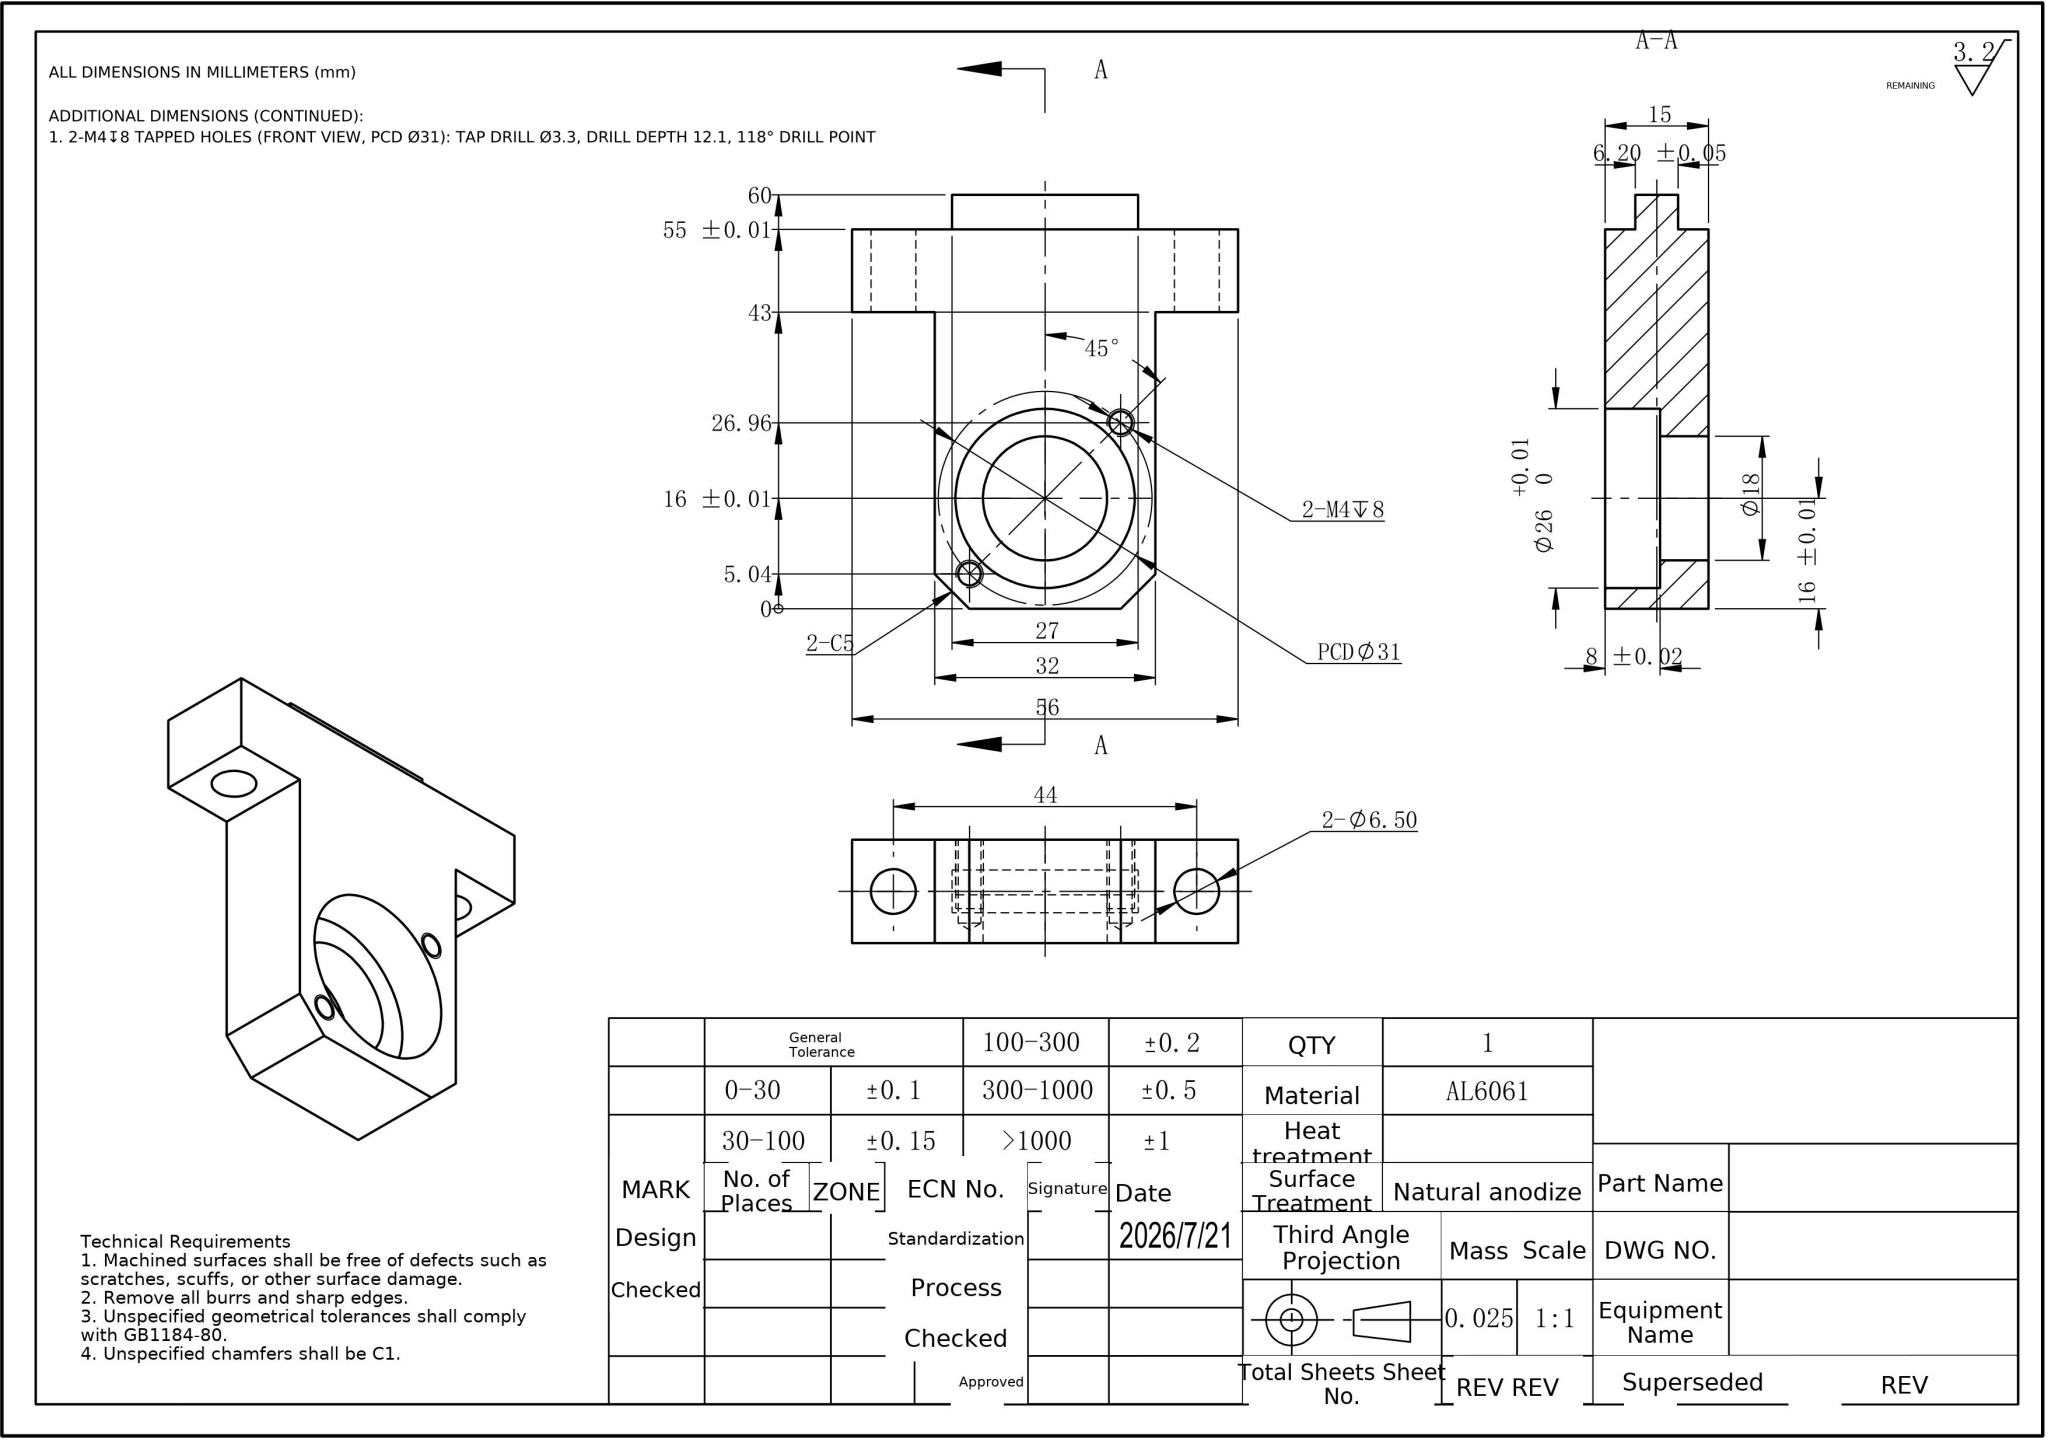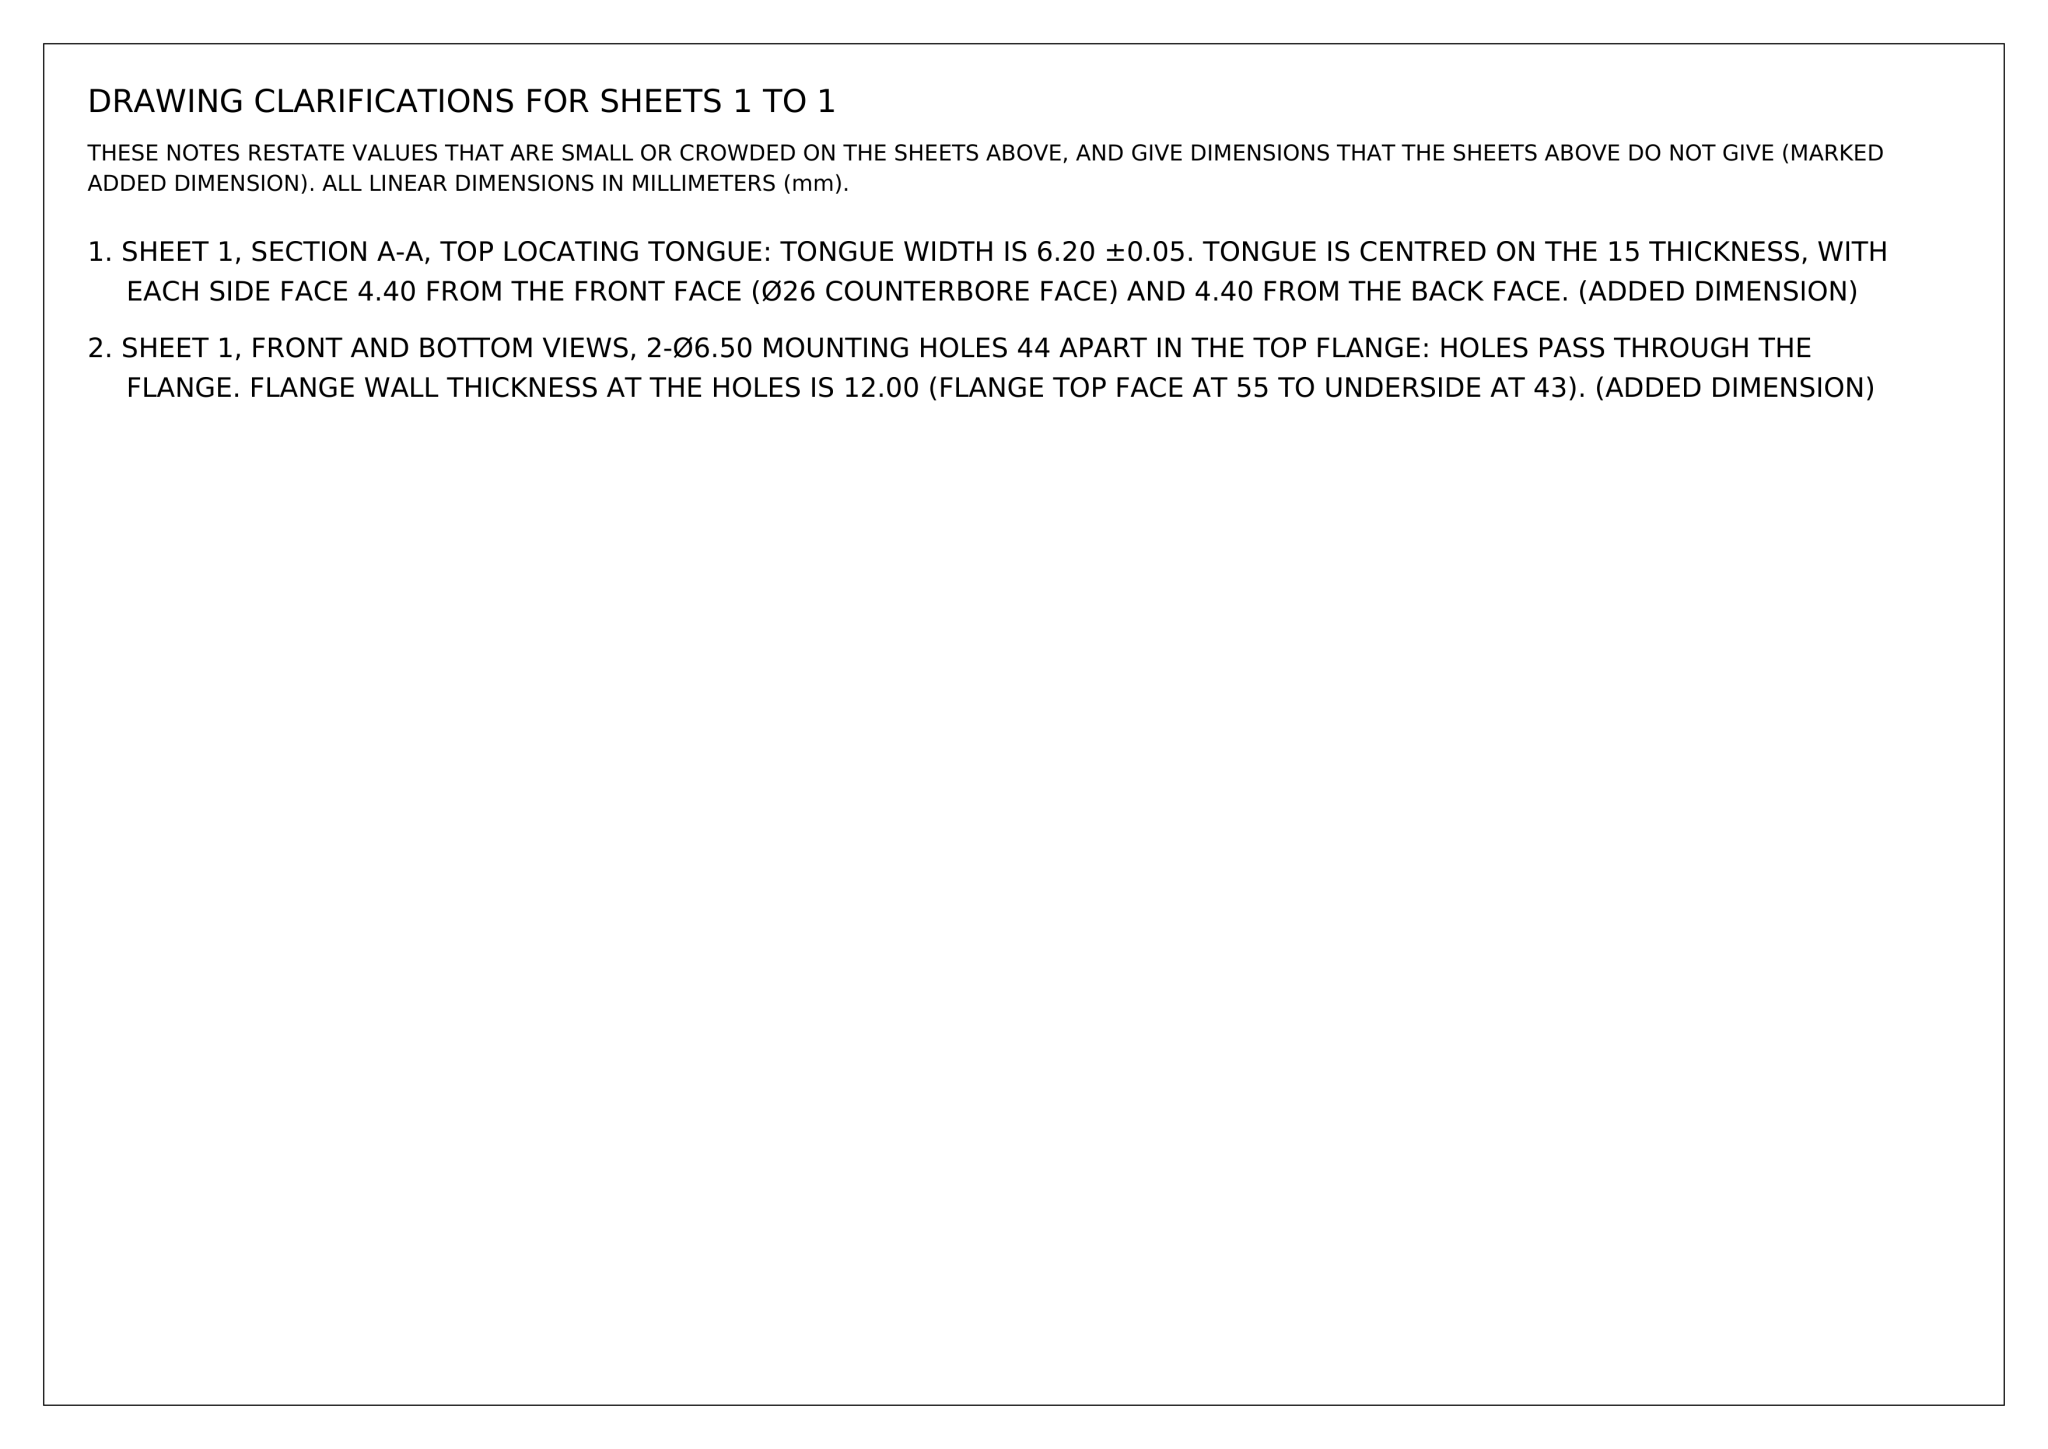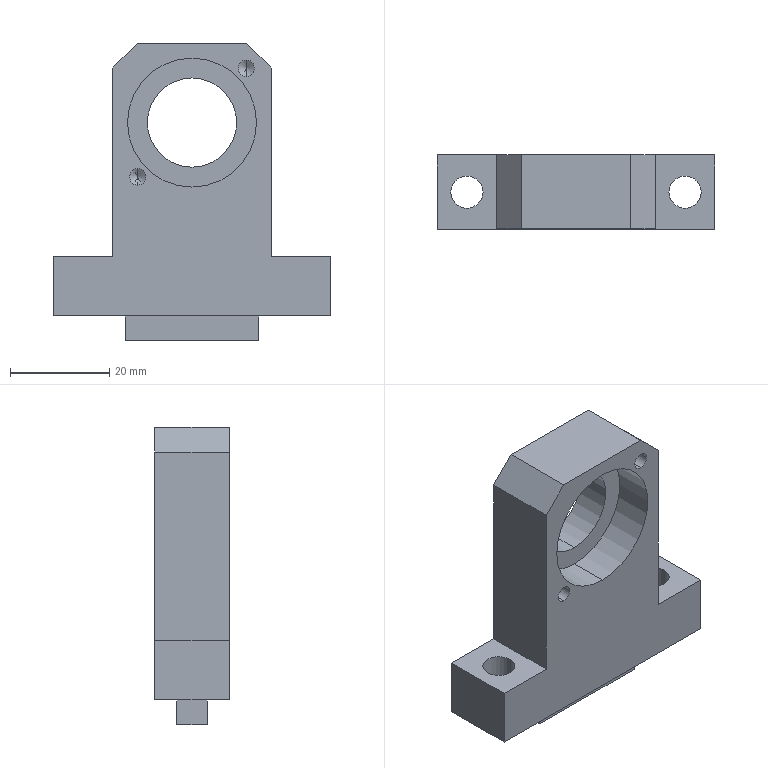Part | NX | mm | 1 solid | 34 faces | box 56 x 15 x 60 mm | volume 24144 mm3 | plane 18 | cylinder 12 | cone 4 | commonest cylinder face diameters 3.3 x4 6.5 x4 26 x2 18 x2